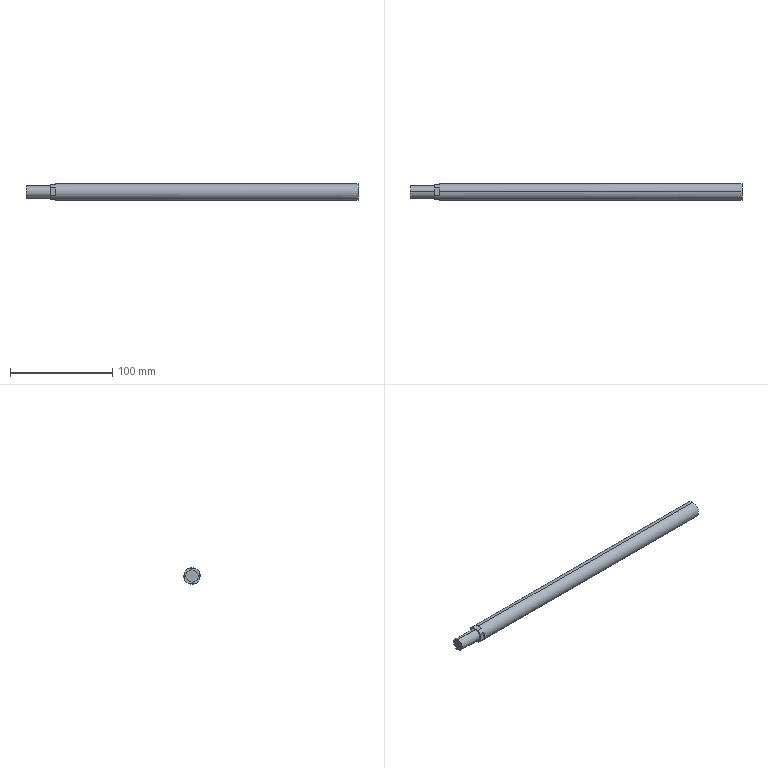Component | SolidWorks | SC40-200PistonRod-1 | 1 solid | 15 faces | box 324 x 16 x 16 mm | volume 62928 mm3 | plane 11 | cylinder 4 | commonest cylinder face diameters 12 x2 16 x2 | material Plain Carbon Steel
STEP:
#1=COLOUR_RGB('',0.7922,0.8196,0.9333);
#2=FILL_AREA_STYLE_COLOUR('',#1);
#3=FILL_AREA_STYLE('',(#2));
#4=SURFACE_STYLE_FILL_AREA(#3);
#5=SURFACE_SIDE_STYLE('',(#4));
#6=SURFACE_STYLE_USAGE(.BOTH.,#5);
#7=PRESENTATION_STYLE_ASSIGNMENT((#6));
#8=CARTESIAN_POINT('',(35.352,51.174,27.288));
#9=VERTEX_POINT('',#8);
#10=CARTESIAN_POINT('',(35.352,51.165,26.816));
#11=VERTEX_POINT('',#10);
#12=CARTESIAN_POINT('',(35.352,51.17,27.052));
#13=DIRECTION('',(-1.,-0.,-0.));
#14=DIRECTION('',(0.,0.01754,0.9998));
#15=AXIS2_PLACEMENT_3D('',#12,#13,#14);
#16=CIRCLE('',#15,0.2362);
#17=EDGE_CURVE('',#9,#11,#16,.T.);
#18=ORIENTED_EDGE('',*,*,#17,.F.);
#19=CARTESIAN_POINT('',(36.297,51.174,27.288));
#20=VERTEX_POINT('',#19);
#21=CARTESIAN_POINT('',(35.352,51.174,27.288));
#22=DIRECTION('',(1.,0.,0.));
#23=VECTOR('',#22,39.37);
#24=LINE('',#21,#23);
#25=EDGE_CURVE('',#9,#20,#24,.T.);
#26=ORIENTED_EDGE('',*,*,#25,.T.);
#27=CARTESIAN_POINT('',(36.297,51.165,26.816));
#28=VERTEX_POINT('',#27);
#29=CARTESIAN_POINT('',(36.297,51.17,27.052));
#30=DIRECTION('',(-1.,-0.,-0.));
#31=DIRECTION('',(0.,0.01754,0.9998));
#32=AXIS2_PLACEMENT_3D('',#29,#30,#31);
#33=CIRCLE('',#32,0.2362);
#34=EDGE_CURVE('',#20,#28,#33,.T.);
#35=ORIENTED_EDGE('',*,*,#34,.T.);
#36=CARTESIAN_POINT('',(35.352,51.165,26.816));
#37=DIRECTION('',(1.,0.,0.));
#38=VECTOR('',#37,39.37);
#39=LINE('',#36,#38);
#40=EDGE_CURVE('',#11,#28,#39,.T.);
#41=ORIENTED_EDGE('',*,*,#40,.F.);
#42=EDGE_LOOP('',(#18,#26,#35,#41));
#43=FACE_OUTER_BOUND('',#42,.T.);
#44=CARTESIAN_POINT('',(35.352,51.17,27.052));
#45=DIRECTION('',(1.,0.,0.));
#46=DIRECTION('',(0.,-0.01754,-0.9998));
#47=AXIS2_PLACEMENT_3D('',#44,#45,#46);
#48=CYLINDRICAL_SURFACE('',#47,0.2362);
#49=ADVANCED_FACE('',(#43),#48,.T.);
#50=CARTESIAN_POINT('',(36.494,51.175,27.367));
#51=VERTEX_POINT('',#50);
#52=CARTESIAN_POINT('',(36.494,51.327,27.325));
#53=VERTEX_POINT('',#52);
#54=CARTESIAN_POINT('',(36.494,51.17,27.052));
#55=DIRECTION('',(-1.,-0.,-0.));
#56=DIRECTION('',(0.,0.01754,0.9998));
#57=AXIS2_PLACEMENT_3D('',#54,#55,#56);
#58=CIRCLE('',#57,0.315);
#59=EDGE_CURVE('',#51,#53,#58,.T.);
#60=ORIENTED_EDGE('',*,*,#59,.F.);
#61=CARTESIAN_POINT('',(48.108,51.175,27.367));
#62=VERTEX_POINT('',#61);
#63=CARTESIAN_POINT('',(36.297,51.175,27.367));
#64=DIRECTION('',(1.,0.,0.));
#65=VECTOR('',#64,39.37);
#66=LINE('',#63,#65);
#67=EDGE_CURVE('',#51,#62,#66,.T.);
#68=ORIENTED_EDGE('',*,*,#67,.T.);
#69=CARTESIAN_POINT('',(48.108,51.164,26.737));
#70=VERTEX_POINT('',#69);
#71=CARTESIAN_POINT('',(48.108,51.17,27.052));
#72=DIRECTION('',(-1.,-0.,-0.));
#73=DIRECTION('',(0.,0.01754,0.9998));
#74=AXIS2_PLACEMENT_3D('',#71,#72,#73);
#75=CIRCLE('',#74,0.315);
#76=EDGE_CURVE('',#62,#70,#75,.T.);
#77=ORIENTED_EDGE('',*,*,#76,.T.);
#78=CARTESIAN_POINT('',(36.494,51.164,26.737));
#79=VERTEX_POINT('',#78);
#80=CARTESIAN_POINT('',(36.297,51.164,26.737));
#81=DIRECTION('',(1.,0.,0.));
#82=VECTOR('',#81,39.37);
#83=LINE('',#80,#82);
#84=EDGE_CURVE('',#79,#70,#83,.T.);
#85=ORIENTED_EDGE('',*,*,#84,.F.);
#86=CARTESIAN_POINT('',(36.494,51.317,26.774));
#87=VERTEX_POINT('',#86);
#88=CARTESIAN_POINT('',(36.494,51.17,27.052));
#89=DIRECTION('',(-1.,-0.,-0.));
#90=DIRECTION('',(0.,0.01754,0.9998));
#91=AXIS2_PLACEMENT_3D('',#88,#89,#90);
#92=CIRCLE('',#91,0.315);
#93=EDGE_CURVE('',#87,#79,#92,.T.);
#94=ORIENTED_EDGE('',*,*,#93,.F.);
#95=CARTESIAN_POINT('',(36.297,51.317,26.774));
#96=VERTEX_POINT('',#95);
#97=CARTESIAN_POINT('',(36.297,51.317,26.774));
#98=DIRECTION('',(1.,0.,0.));
#99=VECTOR('',#98,39.37);
#100=LINE('',#97,#99);
#101=EDGE_CURVE('',#96,#87,#100,.T.);
#102=ORIENTED_EDGE('',*,*,#101,.F.);
#103=CARTESIAN_POINT('',(36.297,51.442,26.895));
#104=VERTEX_POINT('',#103);
#105=CARTESIAN_POINT('',(36.297,51.17,27.052));
#106=DIRECTION('',(-1.,-0.,-0.));
#107=DIRECTION('',(0.,0.01754,0.9998));
#108=AXIS2_PLACEMENT_3D('',#105,#106,#107);
#109=CIRCLE('',#108,0.315);
#110=EDGE_CURVE('',#104,#96,#109,.T.);
#111=ORIENTED_EDGE('',*,*,#110,.F.);
#112=CARTESIAN_POINT('',(36.494,51.442,26.895));
#113=VERTEX_POINT('',#112);
#114=CARTESIAN_POINT('',(36.297,51.442,26.895));
#115=DIRECTION('',(-1.,-0.,-0.));
#116=VECTOR('',#115,39.37);
#117=LINE('',#114,#116);
#118=EDGE_CURVE('',#113,#104,#117,.T.);
#119=ORIENTED_EDGE('',*,*,#118,.F.);
#120=CARTESIAN_POINT('',(36.494,51.448,27.199));
#121=VERTEX_POINT('',#120);
#122=CARTESIAN_POINT('',(36.494,51.17,27.052));
#123=DIRECTION('',(-1.,-0.,-0.));
#124=DIRECTION('',(0.,0.01754,0.9998));
#125=AXIS2_PLACEMENT_3D('',#122,#123,#124);
#126=CIRCLE('',#125,0.315);
#127=EDGE_CURVE('',#121,#113,#126,.T.);
#128=ORIENTED_EDGE('',*,*,#127,.F.);
#129=CARTESIAN_POINT('',(36.297,51.448,27.199));
#130=VERTEX_POINT('',#129);
#131=CARTESIAN_POINT('',(36.297,51.448,27.199));
#132=DIRECTION('',(1.,0.,0.));
#133=VECTOR('',#132,39.37);
#134=LINE('',#131,#133);
#135=EDGE_CURVE('',#130,#121,#134,.T.);
#136=ORIENTED_EDGE('',*,*,#135,.F.);
#137=CARTESIAN_POINT('',(36.297,51.327,27.325));
#138=VERTEX_POINT('',#137);
#139=CARTESIAN_POINT('',(36.297,51.17,27.052));
#140=DIRECTION('',(-1.,-0.,-0.));
#141=DIRECTION('',(0.,0.01754,0.9998));
#142=AXIS2_PLACEMENT_3D('',#139,#140,#141);
#143=CIRCLE('',#142,0.315);
#144=EDGE_CURVE('',#138,#130,#143,.T.);
#145=ORIENTED_EDGE('',*,*,#144,.F.);
#146=CARTESIAN_POINT('',(36.297,51.327,27.325));
#147=DIRECTION('',(-1.,-0.,-0.));
#148=VECTOR('',#147,39.37);
#149=LINE('',#146,#148);
#150=EDGE_CURVE('',#53,#138,#149,.T.);
#151=ORIENTED_EDGE('',*,*,#150,.F.);
#152=EDGE_LOOP('',(#60,#68,#77,#85,#94,#102,#111,#119,#128,#136,#145,#151));
#153=FACE_OUTER_BOUND('',#152,.T.);
#154=CARTESIAN_POINT('',(36.297,51.17,27.052));
#155=DIRECTION('',(1.,0.,0.));
#156=DIRECTION('',(0.,-0.01754,-0.9998));
#157=AXIS2_PLACEMENT_3D('',#154,#155,#156);
#158=CYLINDRICAL_SURFACE('',#157,0.315);
#159=ADVANCED_FACE('',(#153),#158,.T.);
#160=ORIENTED_EDGE('',*,*,#67,.F.);
#161=CARTESIAN_POINT('',(36.494,51.022,27.33));
#162=VERTEX_POINT('',#161);
#163=CARTESIAN_POINT('',(36.494,51.17,27.052));
#164=DIRECTION('',(-1.,-0.,-0.));
#165=DIRECTION('',(0.,0.01754,0.9998));
#166=AXIS2_PLACEMENT_3D('',#163,#164,#165);
#167=CIRCLE('',#166,0.315);
#168=EDGE_CURVE('',#162,#51,#167,.T.);
#169=ORIENTED_EDGE('',*,*,#168,.F.);
#170=CARTESIAN_POINT('',(36.297,51.022,27.33));
#171=VERTEX_POINT('',#170);
#172=CARTESIAN_POINT('',(36.297,51.022,27.33));
#173=DIRECTION('',(1.,0.,0.));
#174=VECTOR('',#173,39.37);
#175=LINE('',#172,#174);
#176=EDGE_CURVE('',#171,#162,#175,.T.);
#177=ORIENTED_EDGE('',*,*,#176,.F.);
#178=CARTESIAN_POINT('',(36.297,50.897,27.209));
#179=VERTEX_POINT('',#178);
#180=CARTESIAN_POINT('',(36.297,51.17,27.052));
#181=DIRECTION('',(-1.,-0.,-0.));
#182=DIRECTION('',(0.,0.01754,0.9998));
#183=AXIS2_PLACEMENT_3D('',#180,#181,#182);
#184=CIRCLE('',#183,0.315);
#185=EDGE_CURVE('',#179,#171,#184,.T.);
#186=ORIENTED_EDGE('',*,*,#185,.F.);
#187=CARTESIAN_POINT('',(36.494,50.897,27.209));
#188=VERTEX_POINT('',#187);
#189=CARTESIAN_POINT('',(36.297,50.897,27.209));
#190=DIRECTION('',(-1.,-0.,-0.));
#191=VECTOR('',#190,39.37);
#192=LINE('',#189,#191);
#193=EDGE_CURVE('',#188,#179,#192,.T.);
#194=ORIENTED_EDGE('',*,*,#193,.F.);
#195=CARTESIAN_POINT('',(36.494,50.891,26.904));
#196=VERTEX_POINT('',#195);
#197=CARTESIAN_POINT('',(36.494,51.17,27.052));
#198=DIRECTION('',(-1.,-0.,-0.));
#199=DIRECTION('',(0.,0.01754,0.9998));
#200=AXIS2_PLACEMENT_3D('',#197,#198,#199);
#201=CIRCLE('',#200,0.315);
#202=EDGE_CURVE('',#196,#188,#201,.T.);
#203=ORIENTED_EDGE('',*,*,#202,.F.);
#204=CARTESIAN_POINT('',(36.297,50.891,26.904));
#205=VERTEX_POINT('',#204);
#206=CARTESIAN_POINT('',(36.297,50.891,26.904));
#207=DIRECTION('',(1.,0.,0.));
#208=VECTOR('',#207,39.37);
#209=LINE('',#206,#208);
#210=EDGE_CURVE('',#205,#196,#209,.T.);
#211=ORIENTED_EDGE('',*,*,#210,.F.);
#212=CARTESIAN_POINT('',(36.297,51.012,26.779));
#213=VERTEX_POINT('',#212);
#214=CARTESIAN_POINT('',(36.297,51.17,27.052));
#215=DIRECTION('',(-1.,-0.,-0.));
#216=DIRECTION('',(0.,0.01754,0.9998));
#217=AXIS2_PLACEMENT_3D('',#214,#215,#216);
#218=CIRCLE('',#217,0.315);
#219=EDGE_CURVE('',#213,#205,#218,.T.);
#220=ORIENTED_EDGE('',*,*,#219,.F.);
#221=CARTESIAN_POINT('',(36.494,51.012,26.779));
#222=VERTEX_POINT('',#221);
#223=CARTESIAN_POINT('',(36.297,51.012,26.779));
#224=DIRECTION('',(-1.,-0.,-0.));
#225=VECTOR('',#224,39.37);
#226=LINE('',#223,#225);
#227=EDGE_CURVE('',#222,#213,#226,.T.);
#228=ORIENTED_EDGE('',*,*,#227,.F.);
#229=CARTESIAN_POINT('',(36.494,51.17,27.052));
#230=DIRECTION('',(-1.,-0.,-0.));
#231=DIRECTION('',(0.,0.01754,0.9998));
#232=AXIS2_PLACEMENT_3D('',#229,#230,#231);
#233=CIRCLE('',#232,0.315);
#234=EDGE_CURVE('',#79,#222,#233,.T.);
#235=ORIENTED_EDGE('',*,*,#234,.F.);
#236=ORIENTED_EDGE('',*,*,#84,.T.);
#237=CARTESIAN_POINT('',(48.108,51.17,27.052));
#238=DIRECTION('',(-1.,-0.,-0.));
#239=DIRECTION('',(0.,0.01754,0.9998));
#240=AXIS2_PLACEMENT_3D('',#237,#238,#239);
#241=CIRCLE('',#240,0.315);
#242=EDGE_CURVE('',#70,#62,#241,.T.);
#243=ORIENTED_EDGE('',*,*,#242,.T.);
#244=EDGE_LOOP('',(#160,#169,#177,#186,#194,#203,#211,#220,#228,#235,#236,#243));
#245=FACE_OUTER_BOUND('',#244,.T.);
#246=CARTESIAN_POINT('',(36.297,51.17,27.052));
#247=DIRECTION('',(1.,0.,0.));
#248=DIRECTION('',(0.,-0.01754,-0.9998));
#249=AXIS2_PLACEMENT_3D('',#246,#247,#248);
#250=CYLINDRICAL_SURFACE('',#249,0.315);
#251=ADVANCED_FACE('',(#245),#250,.T.);
#252=CARTESIAN_POINT('',(36.297,51.17,27.052));
#253=DIRECTION('',(-1.,-0.,-0.));
#254=DIRECTION('',(0.,0.01754,0.9998));
#255=AXIS2_PLACEMENT_3D('',#252,#253,#254);
#256=CIRCLE('',#255,0.2362);
#257=EDGE_CURVE('',#28,#20,#256,.T.);
#258=ORIENTED_EDGE('',*,*,#257,.F.);
#259=ORIENTED_EDGE('',*,*,#34,.F.);
#260=EDGE_LOOP('',(#258,#259));
#261=FACE_BOUND('',#260,.T.);
#262=ORIENTED_EDGE('',*,*,#185,.T.);
#263=CARTESIAN_POINT('',(36.297,51.174,27.327));
#264=DIRECTION('',(-0.,0.9998,-0.01754));
#265=VECTOR('',#264,39.37);
#266=LINE('',#263,#265);
#267=EDGE_CURVE('',#171,#138,#266,.T.);
#268=ORIENTED_EDGE('',*,*,#267,.T.);
#269=ORIENTED_EDGE('',*,*,#144,.T.);
#270=CARTESIAN_POINT('',(36.297,51.445,27.047));
#271=DIRECTION('',(0.,-0.01754,-0.9998));
#272=VECTOR('',#271,39.37);
#273=LINE('',#270,#272);
#274=EDGE_CURVE('',#130,#104,#273,.T.);
#275=ORIENTED_EDGE('',*,*,#274,.T.);
#276=ORIENTED_EDGE('',*,*,#110,.T.);
#277=CARTESIAN_POINT('',(36.297,51.165,26.776));
#278=DIRECTION('',(0.,-0.9998,0.01754));
#279=VECTOR('',#278,39.37);
#280=LINE('',#277,#279);
#281=EDGE_CURVE('',#96,#213,#280,.T.);
#282=ORIENTED_EDGE('',*,*,#281,.T.);
#283=ORIENTED_EDGE('',*,*,#219,.T.);
#284=CARTESIAN_POINT('',(36.297,50.894,27.057));
#285=DIRECTION('',(-0.,0.01754,0.9998));
#286=VECTOR('',#285,39.37);
#287=LINE('',#284,#286);
#288=EDGE_CURVE('',#205,#179,#287,.T.);
#289=ORIENTED_EDGE('',*,*,#288,.T.);
#290=EDGE_LOOP('',(#262,#268,#269,#275,#276,#282,#283,#289));
#291=FACE_OUTER_BOUND('',#290,.T.);
#292=CARTESIAN_POINT('',(36.297,51.17,27.052));
#293=DIRECTION('',(-1.,-0.,-0.));
#294=DIRECTION('',(-0.,0.01754,0.9998));
#295=AXIS2_PLACEMENT_3D('',#292,#293,#294);
#296=PLANE('',#295);
#297=ADVANCED_FACE('',(#261,#291),#296,.T.);
#298=ORIENTED_EDGE('',*,*,#242,.F.);
#299=ORIENTED_EDGE('',*,*,#76,.F.);
#300=EDGE_LOOP('',(#298,#299));
#301=FACE_OUTER_BOUND('',#300,.T.);
#302=CARTESIAN_POINT('',(48.108,51.17,27.052));
#303=DIRECTION('',(-1.,-0.,-0.));
#304=DIRECTION('',(-0.,0.01754,0.9998));
#305=AXIS2_PLACEMENT_3D('',#302,#303,#304);
#306=PLANE('',#305);
#307=ADVANCED_FACE('',(#301),#306,.F.);
#308=ORIENTED_EDGE('',*,*,#25,.F.);
#309=CARTESIAN_POINT('',(35.352,51.17,27.052));
#310=DIRECTION('',(-1.,-0.,-0.));
#311=DIRECTION('',(0.,0.01754,0.9998));
#312=AXIS2_PLACEMENT_3D('',#309,#310,#311);
#313=CIRCLE('',#312,0.2362);
#314=EDGE_CURVE('',#11,#9,#313,.T.);
#315=ORIENTED_EDGE('',*,*,#314,.F.);
#316=ORIENTED_EDGE('',*,*,#40,.T.);
#317=ORIENTED_EDGE('',*,*,#257,.T.);
#318=EDGE_LOOP('',(#308,#315,#316,#317));
#319=FACE_OUTER_BOUND('',#318,.T.);
#320=CARTESIAN_POINT('',(35.352,51.17,27.052));
#321=DIRECTION('',(1.,0.,0.));
#322=DIRECTION('',(0.,-0.01754,-0.9998));
#323=AXIS2_PLACEMENT_3D('',#320,#321,#322);
#324=CYLINDRICAL_SURFACE('',#323,0.2362);
#325=ADVANCED_FACE('',(#319),#324,.T.);
#326=ORIENTED_EDGE('',*,*,#314,.T.);
#327=ORIENTED_EDGE('',*,*,#17,.T.);
#328=EDGE_LOOP('',(#326,#327));
#329=FACE_OUTER_BOUND('',#328,.T.);
#330=CARTESIAN_POINT('',(35.352,51.17,27.052));
#331=DIRECTION('',(-1.,-0.,-0.));
#332=DIRECTION('',(-0.,0.01754,0.9998));
#333=AXIS2_PLACEMENT_3D('',#330,#331,#332);
#334=PLANE('',#333);
#335=ADVANCED_FACE('',(#329),#334,.T.);
#336=ORIENTED_EDGE('',*,*,#135,.T.);
#337=CARTESIAN_POINT('',(36.494,51.44,26.771));
#338=DIRECTION('',(0.,-0.01754,-0.9998));
#339=VECTOR('',#338,39.37);
#340=LINE('',#337,#339);
#341=EDGE_CURVE('',#121,#113,#340,.T.);
#342=ORIENTED_EDGE('',*,*,#341,.T.);
#343=ORIENTED_EDGE('',*,*,#118,.T.);
#344=ORIENTED_EDGE('',*,*,#274,.F.);
#345=EDGE_LOOP('',(#336,#342,#343,#344));
#346=FACE_OUTER_BOUND('',#345,.T.);
#347=CARTESIAN_POINT('',(36.494,51.44,26.771));
#348=DIRECTION('',(-0.,0.9998,-0.01754));
#349=DIRECTION('',(-1.,-0.,-0.));
#350=AXIS2_PLACEMENT_3D('',#347,#348,#349);
#351=PLANE('',#350);
#352=ADVANCED_FACE('',(#346),#351,.T.);
#353=ORIENTED_EDGE('',*,*,#127,.T.);
#354=ORIENTED_EDGE('',*,*,#341,.F.);
#355=EDGE_LOOP('',(#353,#354));
#356=FACE_OUTER_BOUND('',#355,.T.);
#357=CARTESIAN_POINT('',(36.494,51.17,27.052));
#358=DIRECTION('',(-1.,-0.,-0.));
#359=DIRECTION('',(-0.,0.01754,0.9998));
#360=AXIS2_PLACEMENT_3D('',#357,#358,#359);
#361=PLANE('',#360);
#362=ADVANCED_FACE('',(#356),#361,.T.);
#363=ORIENTED_EDGE('',*,*,#101,.T.);
#364=CARTESIAN_POINT('',(36.494,51.44,26.771));
#365=DIRECTION('',(0.,-0.9998,0.01754));
#366=VECTOR('',#365,39.37);
#367=LINE('',#364,#366);
#368=EDGE_CURVE('',#87,#222,#367,.T.);
#369=ORIENTED_EDGE('',*,*,#368,.T.);
#370=ORIENTED_EDGE('',*,*,#227,.T.);
#371=ORIENTED_EDGE('',*,*,#281,.F.);
#372=EDGE_LOOP('',(#363,#369,#370,#371));
#373=FACE_OUTER_BOUND('',#372,.T.);
#374=CARTESIAN_POINT('',(36.494,51.44,26.771));
#375=DIRECTION('',(0.,-0.01754,-0.9998));
#376=DIRECTION('',(0.,-0.9998,0.01754));
#377=AXIS2_PLACEMENT_3D('',#374,#375,#376);
#378=PLANE('',#377);
#379=ADVANCED_FACE('',(#373),#378,.T.);
#380=ORIENTED_EDGE('',*,*,#93,.T.);
#381=ORIENTED_EDGE('',*,*,#234,.T.);
#382=ORIENTED_EDGE('',*,*,#368,.F.);
#383=EDGE_LOOP('',(#380,#381,#382));
#384=FACE_OUTER_BOUND('',#383,.T.);
#385=CARTESIAN_POINT('',(36.494,51.17,27.052));
#386=DIRECTION('',(-1.,-0.,-0.));
#387=DIRECTION('',(-0.,0.01754,0.9998));
#388=AXIS2_PLACEMENT_3D('',#385,#386,#387);
#389=PLANE('',#388);
#390=ADVANCED_FACE('',(#384),#389,.T.);
#391=ORIENTED_EDGE('',*,*,#210,.T.);
#392=CARTESIAN_POINT('',(36.494,50.889,26.781));
#393=DIRECTION('',(-0.,0.01754,0.9998));
#394=VECTOR('',#393,39.37);
#395=LINE('',#392,#394);
#396=EDGE_CURVE('',#196,#188,#395,.T.);
#397=ORIENTED_EDGE('',*,*,#396,.T.);
#398=ORIENTED_EDGE('',*,*,#193,.T.);
#399=ORIENTED_EDGE('',*,*,#288,.F.);
#400=EDGE_LOOP('',(#391,#397,#398,#399));
#401=FACE_OUTER_BOUND('',#400,.T.);
#402=CARTESIAN_POINT('',(36.494,50.889,26.781));
#403=DIRECTION('',(0.,-0.9998,0.01754));
#404=DIRECTION('',(1.,0.,0.));
#405=AXIS2_PLACEMENT_3D('',#402,#403,#404);
#406=PLANE('',#405);
#407=ADVANCED_FACE('',(#401),#406,.T.);
#408=ORIENTED_EDGE('',*,*,#202,.T.);
#409=ORIENTED_EDGE('',*,*,#396,.F.);
#410=EDGE_LOOP('',(#408,#409));
#411=FACE_OUTER_BOUND('',#410,.T.);
#412=CARTESIAN_POINT('',(36.494,51.17,27.052));
#413=DIRECTION('',(-1.,-0.,-0.));
#414=DIRECTION('',(-0.,0.01754,0.9998));
#415=AXIS2_PLACEMENT_3D('',#412,#413,#414);
#416=PLANE('',#415);
#417=ADVANCED_FACE('',(#411),#416,.T.);
#418=ORIENTED_EDGE('',*,*,#168,.T.);
#419=ORIENTED_EDGE('',*,*,#59,.T.);
#420=CARTESIAN_POINT('',(36.494,51.45,27.323));
#421=DIRECTION('',(-0.,0.9998,-0.01754));
#422=VECTOR('',#421,39.37);
#423=LINE('',#420,#422);
#424=EDGE_CURVE('',#162,#53,#423,.T.);
#425=ORIENTED_EDGE('',*,*,#424,.F.);
#426=EDGE_LOOP('',(#418,#419,#425));
#427=FACE_OUTER_BOUND('',#426,.T.);
#428=CARTESIAN_POINT('',(36.494,51.17,27.052));
#429=DIRECTION('',(-1.,-0.,-0.));
#430=DIRECTION('',(-0.,0.01754,0.9998));
#431=AXIS2_PLACEMENT_3D('',#428,#429,#430);
#432=PLANE('',#431);
#433=ADVANCED_FACE('',(#427),#432,.T.);
#434=ORIENTED_EDGE('',*,*,#176,.T.);
#435=ORIENTED_EDGE('',*,*,#424,.T.);
#436=ORIENTED_EDGE('',*,*,#150,.T.);
#437=ORIENTED_EDGE('',*,*,#267,.F.);
#438=EDGE_LOOP('',(#434,#435,#436,#437));
#439=FACE_OUTER_BOUND('',#438,.T.);
#440=CARTESIAN_POINT('',(36.494,51.45,27.323));
#441=DIRECTION('',(-0.,0.01754,0.9998));
#442=DIRECTION('',(-0.,0.9998,-0.01754));
#443=AXIS2_PLACEMENT_3D('',#440,#441,#442);
#444=PLANE('',#443);
#445=ADVANCED_FACE('',(#439),#444,.T.);
#446=CLOSED_SHELL('',(#49,#159,#251,#297,#307,#325,#335,#352,#362,#379,#390,#407,#417,#433,#445));
#447=MANIFOLD_SOLID_BREP('',#446);
#448=STYLED_ITEM('',(#7),#447);
#449=PRESENTATION_LAYER_ASSIGNMENT('','',(#448));
#450=(LENGTH_UNIT()NAMED_UNIT(*)SI_UNIT($,.METRE.));
#451=LENGTH_MEASURE_WITH_UNIT(LENGTH_MEASURE(0.0254),#450);
#452=DIMENSIONAL_EXPONENTS(1.,0.,0.,0.,0.,0.,0.);
#453=(CONVERSION_BASED_UNIT('',#451)LENGTH_UNIT()NAMED_UNIT(#452));
#454=UNCERTAINTY_MEASURE_WITH_UNIT(LENGTH_MEASURE(0.00001),#453,'','');
#455=(NAMED_UNIT(*)PLANE_ANGLE_UNIT()SI_UNIT($,.RADIAN.));
#456=(NAMED_UNIT(*)SI_UNIT($,.STERADIAN.)SOLID_ANGLE_UNIT());
#457=(GEOMETRIC_REPRESENTATION_CONTEXT(3)GLOBAL_UNCERTAINTY_ASSIGNED_CONTEXT((#454))GLOBAL_UNIT_ASSIGNED_CONTEXT((#453,#455,#456))REPRESENTATION_CONTEXT('',''));
#458=MECHANICAL_DESIGN_GEOMETRIC_PRESENTATION_REPRESENTATION('',(#448),#457);
#459=CARTESIAN_POINT('',(0.,0.,0.));
#460=DIRECTION('',(0.,0.,1.));
#461=DIRECTION('',(1.,0.,0.));
#462=AXIS2_PLACEMENT_3D('',#459,#460,#461);
#463=(LENGTH_UNIT()NAMED_UNIT(*)SI_UNIT($,.METRE.));
#464=LENGTH_MEASURE_WITH_UNIT(LENGTH_MEASURE(0.0254),#463);
#465=DIMENSIONAL_EXPONENTS(1.,0.,0.,0.,0.,0.,0.);
#466=(CONVERSION_BASED_UNIT('',#464)LENGTH_UNIT()NAMED_UNIT(#465));
#467=UNCERTAINTY_MEASURE_WITH_UNIT(LENGTH_MEASURE(0.00001),#466,'','');
#468=(NAMED_UNIT(*)PLANE_ANGLE_UNIT()SI_UNIT($,.RADIAN.));
#469=(NAMED_UNIT(*)SI_UNIT($,.STERADIAN.)SOLID_ANGLE_UNIT());
#470=(GEOMETRIC_REPRESENTATION_CONTEXT(3)GLOBAL_UNCERTAINTY_ASSIGNED_CONTEXT((#467))GLOBAL_UNIT_ASSIGNED_CONTEXT((#466,#468,#469))REPRESENTATION_CONTEXT('',''));
#471=ADVANCED_BREP_SHAPE_REPRESENTATION('',(#447,#462),#470);